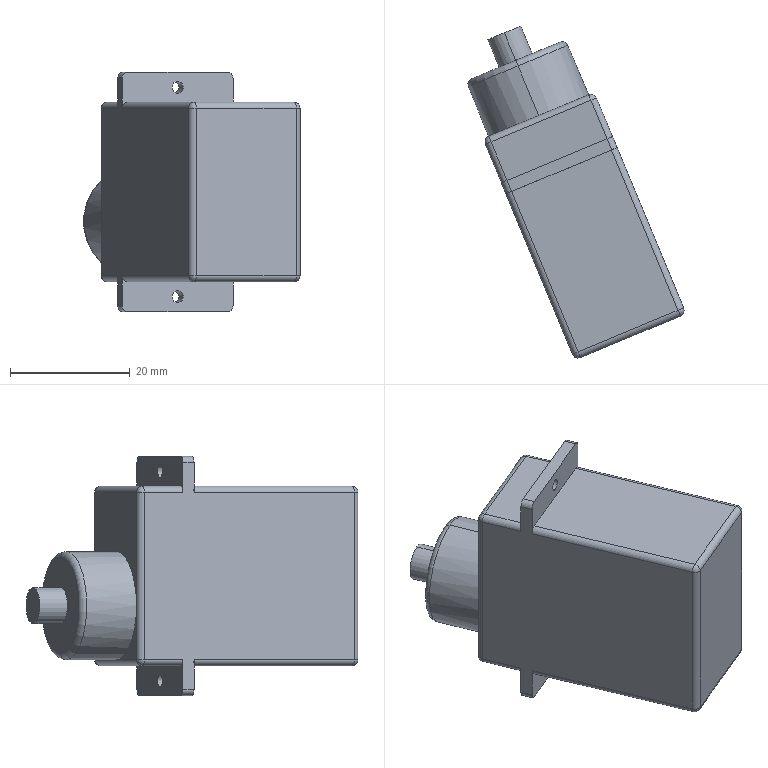Component | SolidWorks | SteeringController-1 | 1 solid | 55 faces | volume 27121 mm3 | cylinder 28 | plane 17 | sphere 8 | torus 2 | commonest cylinder face diameters 2 x24 6 x2 18.09 x2